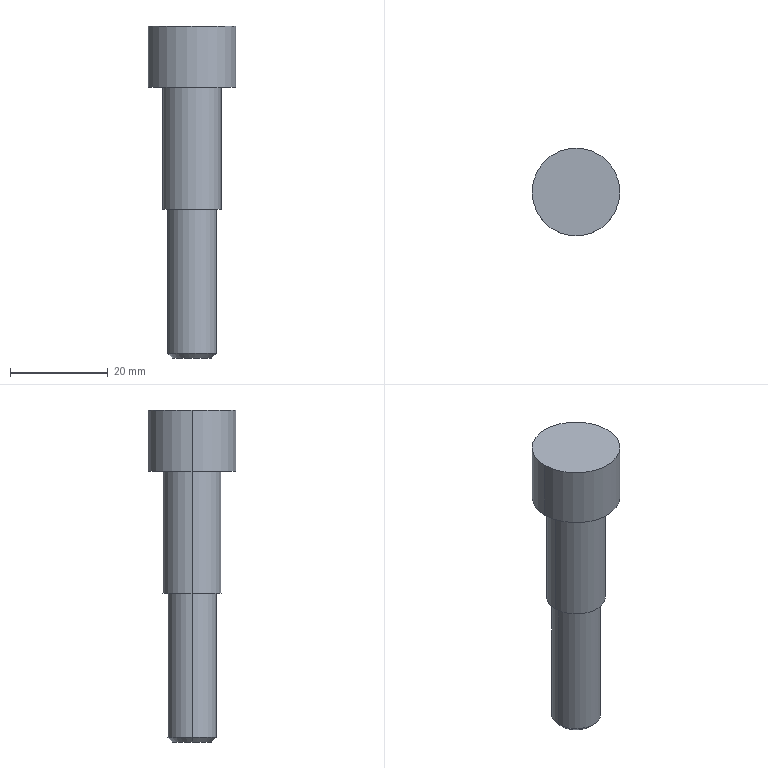Component | SolidWorks | ScrewM10-1 | 1 solid | 12 faces | box 18 x 18 x 68 mm | volume 8389 mm3 | cylinder 6 | plane 4 | cone 2 | commonest cylinder face diameters 10 x2 12 x2 18 x2
build123d program:
from build123d import *

# Parameters (mm, degrees)
CHAMFER1_SIZE = 1


with BuildPart() as part:
    # Sketch1 → Revolve1 (revolve)
    with BuildSketch(Plane.XY, mode=Mode.PRIVATE) as revolve1_sk:
        Polygon((0, 0), (9, 0), (9, 12.5), (6, 12.5), (6, 37.5), (5, 37.5), (5, 68), (0, 68), align=None)
    revolve(revolve1_sk.sketch.rotate(Axis((0, 68, 0), (0, -1, 0)), 180), axis=Axis((0, 68, 0), (0, -1, 0)))

    # Chamfer1
    chamfer1_edges = [part.edges().sort_by_distance(p)[0] for p in [
        (5, 68, 0),
    ]]
    chamfer(chamfer1_edges, length=CHAMFER1_SIZE)


solid = part.part

# Placed as in the assembly
solid = solid.moved(Location((-60.871, 27.262, 12.561), (-90, 0, 0)))
STEP:
#1=CARTESIAN_POINT('',(-2.554,1.073,-2.183));
#2=VERTEX_POINT('',#1);
#3=CARTESIAN_POINT('',(-2.239,1.073,-2.183));
#4=VERTEX_POINT('',#3);
#5=CARTESIAN_POINT('',(-2.396,1.073,-2.183));
#6=DIRECTION('',(0.,-0.,-1.));
#7=DIRECTION('',(1.,0.,0.));
#8=AXIS2_PLACEMENT_3D('',#5,#6,#7);
#9=CIRCLE('',#8,0.1575);
#10=EDGE_CURVE('',#2,#4,#9,.T.);
#11=ORIENTED_EDGE('',*,*,#10,.F.);
#12=CARTESIAN_POINT('',(-2.593,1.073,-2.143));
#13=VERTEX_POINT('',#12);
#14=CARTESIAN_POINT('',(-2.554,1.073,-2.183));
#15=DIRECTION('',(-0.7071,0.,0.7071));
#16=VECTOR('',#15,39.37);
#17=LINE('',#14,#16);
#18=EDGE_CURVE('',#2,#13,#17,.T.);
#19=ORIENTED_EDGE('',*,*,#18,.T.);
#20=CARTESIAN_POINT('',(-2.2,1.073,-2.143));
#21=VERTEX_POINT('',#20);
#22=CARTESIAN_POINT('',(-2.396,1.073,-2.143));
#23=DIRECTION('',(0.,0.,1.));
#24=DIRECTION('',(1.,0.,0.));
#25=AXIS2_PLACEMENT_3D('',#22,#23,#24);
#26=CIRCLE('',#25,0.1969);
#27=EDGE_CURVE('',#21,#13,#26,.T.);
#28=ORIENTED_EDGE('',*,*,#27,.F.);
#29=CARTESIAN_POINT('',(-2.239,1.073,-2.183));
#30=DIRECTION('',(0.7071,0.,0.7071));
#31=VECTOR('',#30,39.37);
#32=LINE('',#29,#31);
#33=EDGE_CURVE('',#4,#21,#32,.T.);
#34=ORIENTED_EDGE('',*,*,#33,.F.);
#35=EDGE_LOOP('',(#11,#19,#28,#34));
#36=FACE_OUTER_BOUND('',#35,.T.);
#37=CARTESIAN_POINT('',(-2.396,1.073,-2.183));
#38=DIRECTION('',(0.,0.,1.));
#39=DIRECTION('',(1.,0.,0.));
#40=AXIS2_PLACEMENT_3D('',#37,#38,#39);
#41=CONICAL_SURFACE('',#40,0.1575,0.7854);
#42=ADVANCED_FACE('',(#36),#41,.T.);
#43=CARTESIAN_POINT('',(-2.593,1.073,-0.9819));
#44=VERTEX_POINT('',#43);
#45=CARTESIAN_POINT('',(-2.2,1.073,-0.9819));
#46=VERTEX_POINT('',#45);
#47=CARTESIAN_POINT('',(-2.396,1.073,-0.9819));
#48=DIRECTION('',(0.,-0.,-1.));
#49=DIRECTION('',(-1.,0.,0.));
#50=AXIS2_PLACEMENT_3D('',#47,#48,#49);
#51=CIRCLE('',#50,0.1969);
#52=EDGE_CURVE('',#44,#46,#51,.T.);
#53=ORIENTED_EDGE('',*,*,#52,.T.);
#54=CARTESIAN_POINT('',(-2.2,1.073,-2.183));
#55=DIRECTION('',(0.,-0.,-1.));
#56=VECTOR('',#55,39.37);
#57=LINE('',#54,#56);
#58=EDGE_CURVE('',#46,#21,#57,.T.);
#59=ORIENTED_EDGE('',*,*,#58,.T.);
#60=ORIENTED_EDGE('',*,*,#27,.T.);
#61=CARTESIAN_POINT('',(-2.593,1.073,-2.183));
#62=DIRECTION('',(0.,-0.,-1.));
#63=VECTOR('',#62,39.37);
#64=LINE('',#61,#63);
#65=EDGE_CURVE('',#44,#13,#64,.T.);
#66=ORIENTED_EDGE('',*,*,#65,.F.);
#67=EDGE_LOOP('',(#53,#59,#60,#66));
#68=FACE_OUTER_BOUND('',#67,.T.);
#69=CARTESIAN_POINT('',(-2.396,1.073,-2.183));
#70=DIRECTION('',(0.,-0.,-1.));
#71=DIRECTION('',(-1.,0.,0.));
#72=AXIS2_PLACEMENT_3D('',#69,#70,#71);
#73=CYLINDRICAL_SURFACE('',#72,0.1969);
#74=ADVANCED_FACE('',(#68),#73,.T.);
#75=CARTESIAN_POINT('',(-2.633,1.073,0.002394));
#76=VERTEX_POINT('',#75);
#77=CARTESIAN_POINT('',(-2.16,1.073,0.002394));
#78=VERTEX_POINT('',#77);
#79=CARTESIAN_POINT('',(-2.396,1.073,0.002394));
#80=DIRECTION('',(0.,-0.,-1.));
#81=DIRECTION('',(-1.,0.,0.));
#82=AXIS2_PLACEMENT_3D('',#79,#80,#81);
#83=CIRCLE('',#82,0.2362);
#84=EDGE_CURVE('',#76,#78,#83,.T.);
#85=ORIENTED_EDGE('',*,*,#84,.T.);
#86=CARTESIAN_POINT('',(-2.16,1.073,-0.9819));
#87=VERTEX_POINT('',#86);
#88=CARTESIAN_POINT('',(-2.16,1.073,-2.183));
#89=DIRECTION('',(0.,-0.,-1.));
#90=VECTOR('',#89,39.37);
#91=LINE('',#88,#90);
#92=EDGE_CURVE('',#78,#87,#91,.T.);
#93=ORIENTED_EDGE('',*,*,#92,.T.);
#94=CARTESIAN_POINT('',(-2.633,1.073,-0.9819));
#95=VERTEX_POINT('',#94);
#96=CARTESIAN_POINT('',(-2.396,1.073,-0.9819));
#97=DIRECTION('',(0.,-0.,-1.));
#98=DIRECTION('',(-1.,0.,0.));
#99=AXIS2_PLACEMENT_3D('',#96,#97,#98);
#100=CIRCLE('',#99,0.2362);
#101=EDGE_CURVE('',#95,#87,#100,.T.);
#102=ORIENTED_EDGE('',*,*,#101,.F.);
#103=CARTESIAN_POINT('',(-2.633,1.073,-2.183));
#104=DIRECTION('',(0.,-0.,-1.));
#105=VECTOR('',#104,39.37);
#106=LINE('',#103,#105);
#107=EDGE_CURVE('',#76,#95,#106,.T.);
#108=ORIENTED_EDGE('',*,*,#107,.F.);
#109=EDGE_LOOP('',(#85,#93,#102,#108));
#110=FACE_OUTER_BOUND('',#109,.T.);
#111=CARTESIAN_POINT('',(-2.396,1.073,-2.183));
#112=DIRECTION('',(0.,-0.,-1.));
#113=DIRECTION('',(-1.,0.,0.));
#114=AXIS2_PLACEMENT_3D('',#111,#112,#113);
#115=CYLINDRICAL_SURFACE('',#114,0.2362);
#116=ADVANCED_FACE('',(#110),#115,.T.);
#117=CARTESIAN_POINT('',(-2.751,1.073,0.4945));
#118=VERTEX_POINT('',#117);
#119=CARTESIAN_POINT('',(-2.042,1.073,0.4945));
#120=VERTEX_POINT('',#119);
#121=CARTESIAN_POINT('',(-2.396,1.073,0.4945));
#122=DIRECTION('',(0.,-0.,-1.));
#123=DIRECTION('',(-1.,0.,0.));
#124=AXIS2_PLACEMENT_3D('',#121,#122,#123);
#125=CIRCLE('',#124,0.3543);
#126=EDGE_CURVE('',#118,#120,#125,.T.);
#127=ORIENTED_EDGE('',*,*,#126,.T.);
#128=CARTESIAN_POINT('',(-2.042,1.073,0.002394));
#129=VERTEX_POINT('',#128);
#130=CARTESIAN_POINT('',(-2.042,1.073,-2.183));
#131=DIRECTION('',(0.,-0.,-1.));
#132=VECTOR('',#131,39.37);
#133=LINE('',#130,#132);
#134=EDGE_CURVE('',#120,#129,#133,.T.);
#135=ORIENTED_EDGE('',*,*,#134,.T.);
#136=CARTESIAN_POINT('',(-2.751,1.073,0.002394));
#137=VERTEX_POINT('',#136);
#138=CARTESIAN_POINT('',(-2.396,1.073,0.002394));
#139=DIRECTION('',(0.,-0.,-1.));
#140=DIRECTION('',(-1.,0.,0.));
#141=AXIS2_PLACEMENT_3D('',#138,#139,#140);
#142=CIRCLE('',#141,0.3543);
#143=EDGE_CURVE('',#137,#129,#142,.T.);
#144=ORIENTED_EDGE('',*,*,#143,.F.);
#145=CARTESIAN_POINT('',(-2.751,1.073,-2.183));
#146=DIRECTION('',(0.,-0.,-1.));
#147=VECTOR('',#146,39.37);
#148=LINE('',#145,#147);
#149=EDGE_CURVE('',#118,#137,#148,.T.);
#150=ORIENTED_EDGE('',*,*,#149,.F.);
#151=EDGE_LOOP('',(#127,#135,#144,#150));
#152=FACE_OUTER_BOUND('',#151,.T.);
#153=CARTESIAN_POINT('',(-2.396,1.073,-2.183));
#154=DIRECTION('',(0.,-0.,-1.));
#155=DIRECTION('',(-1.,0.,0.));
#156=AXIS2_PLACEMENT_3D('',#153,#154,#155);
#157=CYLINDRICAL_SURFACE('',#156,0.3543);
#158=ADVANCED_FACE('',(#152),#157,.T.);
#159=ORIENTED_EDGE('',*,*,#126,.F.);
#160=CARTESIAN_POINT('',(-2.396,1.073,0.4945));
#161=DIRECTION('',(0.,-0.,-1.));
#162=DIRECTION('',(-1.,0.,0.));
#163=AXIS2_PLACEMENT_3D('',#160,#161,#162);
#164=CIRCLE('',#163,0.3543);
#165=EDGE_CURVE('',#120,#118,#164,.T.);
#166=ORIENTED_EDGE('',*,*,#165,.F.);
#167=EDGE_LOOP('',(#159,#166));
#168=FACE_OUTER_BOUND('',#167,.T.);
#169=CARTESIAN_POINT('',(-2.396,1.073,0.4945));
#170=DIRECTION('',(0.,-0.,-1.));
#171=DIRECTION('',(-1.,-0.,0.));
#172=AXIS2_PLACEMENT_3D('',#169,#170,#171);
#173=PLANE('',#172);
#174=ADVANCED_FACE('',(#168),#173,.F.);
#175=ORIENTED_EDGE('',*,*,#134,.F.);
#176=ORIENTED_EDGE('',*,*,#165,.T.);
#177=ORIENTED_EDGE('',*,*,#149,.T.);
#178=CARTESIAN_POINT('',(-2.396,1.073,0.002394));
#179=DIRECTION('',(0.,-0.,-1.));
#180=DIRECTION('',(-1.,0.,0.));
#181=AXIS2_PLACEMENT_3D('',#178,#179,#180);
#182=CIRCLE('',#181,0.3543);
#183=EDGE_CURVE('',#129,#137,#182,.T.);
#184=ORIENTED_EDGE('',*,*,#183,.F.);
#185=EDGE_LOOP('',(#175,#176,#177,#184));
#186=FACE_OUTER_BOUND('',#185,.T.);
#187=CARTESIAN_POINT('',(-2.396,1.073,-2.183));
#188=DIRECTION('',(0.,-0.,-1.));
#189=DIRECTION('',(-1.,0.,0.));
#190=AXIS2_PLACEMENT_3D('',#187,#188,#189);
#191=CYLINDRICAL_SURFACE('',#190,0.3543);
#192=ADVANCED_FACE('',(#186),#191,.T.);
#193=ORIENTED_EDGE('',*,*,#84,.F.);
#194=CARTESIAN_POINT('',(-2.396,1.073,0.002394));
#195=DIRECTION('',(0.,-0.,-1.));
#196=DIRECTION('',(-1.,0.,0.));
#197=AXIS2_PLACEMENT_3D('',#194,#195,#196);
#198=CIRCLE('',#197,0.2362);
#199=EDGE_CURVE('',#78,#76,#198,.T.);
#200=ORIENTED_EDGE('',*,*,#199,.F.);
#201=EDGE_LOOP('',(#193,#200));
#202=FACE_BOUND('',#201,.T.);
#203=ORIENTED_EDGE('',*,*,#143,.T.);
#204=ORIENTED_EDGE('',*,*,#183,.T.);
#205=EDGE_LOOP('',(#203,#204));
#206=FACE_OUTER_BOUND('',#205,.T.);
#207=CARTESIAN_POINT('',(-2.042,1.073,0.002394));
#208=DIRECTION('',(-0.,0.,1.));
#209=DIRECTION('',(1.,0.,0.));
#210=AXIS2_PLACEMENT_3D('',#207,#208,#209);
#211=PLANE('',#210);
#212=ADVANCED_FACE('',(#202,#206),#211,.F.);
#213=ORIENTED_EDGE('',*,*,#92,.F.);
#214=ORIENTED_EDGE('',*,*,#199,.T.);
#215=ORIENTED_EDGE('',*,*,#107,.T.);
#216=CARTESIAN_POINT('',(-2.396,1.073,-0.9819));
#217=DIRECTION('',(0.,-0.,-1.));
#218=DIRECTION('',(-1.,0.,0.));
#219=AXIS2_PLACEMENT_3D('',#216,#217,#218);
#220=CIRCLE('',#219,0.2362);
#221=EDGE_CURVE('',#87,#95,#220,.T.);
#222=ORIENTED_EDGE('',*,*,#221,.F.);
#223=EDGE_LOOP('',(#213,#214,#215,#222));
#224=FACE_OUTER_BOUND('',#223,.T.);
#225=CARTESIAN_POINT('',(-2.396,1.073,-2.183));
#226=DIRECTION('',(0.,-0.,-1.));
#227=DIRECTION('',(-1.,0.,0.));
#228=AXIS2_PLACEMENT_3D('',#225,#226,#227);
#229=CYLINDRICAL_SURFACE('',#228,0.2362);
#230=ADVANCED_FACE('',(#224),#229,.T.);
#231=ORIENTED_EDGE('',*,*,#52,.F.);
#232=CARTESIAN_POINT('',(-2.396,1.073,-0.9819));
#233=DIRECTION('',(0.,-0.,-1.));
#234=DIRECTION('',(-1.,0.,0.));
#235=AXIS2_PLACEMENT_3D('',#232,#233,#234);
#236=CIRCLE('',#235,0.1969);
#237=EDGE_CURVE('',#46,#44,#236,.T.);
#238=ORIENTED_EDGE('',*,*,#237,.F.);
#239=EDGE_LOOP('',(#231,#238));
#240=FACE_BOUND('',#239,.T.);
#241=ORIENTED_EDGE('',*,*,#101,.T.);
#242=ORIENTED_EDGE('',*,*,#221,.T.);
#243=EDGE_LOOP('',(#241,#242));
#244=FACE_OUTER_BOUND('',#243,.T.);
#245=CARTESIAN_POINT('',(-2.16,1.073,-0.9819));
#246=DIRECTION('',(-0.,0.,1.));
#247=DIRECTION('',(1.,0.,0.));
#248=AXIS2_PLACEMENT_3D('',#245,#246,#247);
#249=PLANE('',#248);
#250=ADVANCED_FACE('',(#240,#244),#249,.F.);
#251=ORIENTED_EDGE('',*,*,#58,.F.);
#252=ORIENTED_EDGE('',*,*,#237,.T.);
#253=ORIENTED_EDGE('',*,*,#65,.T.);
#254=CARTESIAN_POINT('',(-2.396,1.073,-2.143));
#255=DIRECTION('',(0.,0.,1.));
#256=DIRECTION('',(1.,0.,0.));
#257=AXIS2_PLACEMENT_3D('',#254,#255,#256);
#258=CIRCLE('',#257,0.1969);
#259=EDGE_CURVE('',#13,#21,#258,.T.);
#260=ORIENTED_EDGE('',*,*,#259,.T.);
#261=EDGE_LOOP('',(#251,#252,#253,#260));
#262=FACE_OUTER_BOUND('',#261,.T.);
#263=CARTESIAN_POINT('',(-2.396,1.073,-2.183));
#264=DIRECTION('',(0.,-0.,-1.));
#265=DIRECTION('',(-1.,0.,0.));
#266=AXIS2_PLACEMENT_3D('',#263,#264,#265);
#267=CYLINDRICAL_SURFACE('',#266,0.1969);
#268=ADVANCED_FACE('',(#262),#267,.T.);
#269=CARTESIAN_POINT('',(-2.396,1.073,-2.183));
#270=DIRECTION('',(0.,-0.,-1.));
#271=DIRECTION('',(1.,0.,0.));
#272=AXIS2_PLACEMENT_3D('',#269,#270,#271);
#273=CIRCLE('',#272,0.1575);
#274=EDGE_CURVE('',#4,#2,#273,.T.);
#275=ORIENTED_EDGE('',*,*,#274,.T.);
#276=ORIENTED_EDGE('',*,*,#10,.T.);
#277=EDGE_LOOP('',(#275,#276));
#278=FACE_OUTER_BOUND('',#277,.T.);
#279=CARTESIAN_POINT('',(-2.2,1.073,-2.183));
#280=DIRECTION('',(-0.,0.,1.));
#281=DIRECTION('',(1.,0.,0.));
#282=AXIS2_PLACEMENT_3D('',#279,#280,#281);
#283=PLANE('',#282);
#284=ADVANCED_FACE('',(#278),#283,.F.);
#285=ORIENTED_EDGE('',*,*,#18,.F.);
#286=ORIENTED_EDGE('',*,*,#274,.F.);
#287=ORIENTED_EDGE('',*,*,#33,.T.);
#288=ORIENTED_EDGE('',*,*,#259,.F.);
#289=EDGE_LOOP('',(#285,#286,#287,#288));
#290=FACE_OUTER_BOUND('',#289,.T.);
#291=CARTESIAN_POINT('',(-2.396,1.073,-2.183));
#292=DIRECTION('',(0.,0.,1.));
#293=DIRECTION('',(1.,0.,0.));
#294=AXIS2_PLACEMENT_3D('',#291,#292,#293);
#295=CONICAL_SURFACE('',#294,0.1575,0.7854);
#296=ADVANCED_FACE('',(#290),#295,.T.);
#297=CLOSED_SHELL('',(#42,#74,#116,#158,#174,#192,#212,#230,#250,#268,#284,#296));
#298=MANIFOLD_SOLID_BREP('',#297);
#299=CARTESIAN_POINT('',(0.,0.,0.));
#300=DIRECTION('',(0.,0.,1.));
#301=DIRECTION('',(1.,0.,0.));
#302=AXIS2_PLACEMENT_3D('',#299,#300,#301);
#303=(LENGTH_UNIT()NAMED_UNIT(*)SI_UNIT($,.METRE.));
#304=LENGTH_MEASURE_WITH_UNIT(LENGTH_MEASURE(0.0254),#303);
#305=DIMENSIONAL_EXPONENTS(1.,0.,0.,0.,0.,0.,0.);
#306=(CONVERSION_BASED_UNIT('',#304)LENGTH_UNIT()NAMED_UNIT(#305));
#307=UNCERTAINTY_MEASURE_WITH_UNIT(LENGTH_MEASURE(0.00001),#306,'','');
#308=(NAMED_UNIT(*)PLANE_ANGLE_UNIT()SI_UNIT($,.RADIAN.));
#309=(NAMED_UNIT(*)SI_UNIT($,.STERADIAN.)SOLID_ANGLE_UNIT());
#310=(GEOMETRIC_REPRESENTATION_CONTEXT(3)GLOBAL_UNCERTAINTY_ASSIGNED_CONTEXT((#307))GLOBAL_UNIT_ASSIGNED_CONTEXT((#306,#308,#309))REPRESENTATION_CONTEXT('',''));
#311=ADVANCED_BREP_SHAPE_REPRESENTATION('',(#298,#302),#310);
#312=COLOUR_RGB('',0.7922,0.8196,0.9333);
#313=FILL_AREA_STYLE_COLOUR('',#312);
#314=FILL_AREA_STYLE('',(#313));
#315=SURFACE_STYLE_FILL_AREA(#314);
#316=SURFACE_SIDE_STYLE('',(#315));
#317=SURFACE_STYLE_USAGE(.BOTH.,#316);
#318=PRESENTATION_STYLE_ASSIGNMENT((#317));
#319=STYLED_ITEM('',(#318),#298);
#320=(LENGTH_UNIT()NAMED_UNIT(*)SI_UNIT($,.METRE.));
#321=LENGTH_MEASURE_WITH_UNIT(LENGTH_MEASURE(0.0254),#320);
#322=DIMENSIONAL_EXPONENTS(1.,0.,0.,0.,0.,0.,0.);
#323=(CONVERSION_BASED_UNIT('',#321)LENGTH_UNIT()NAMED_UNIT(#322));
#324=UNCERTAINTY_MEASURE_WITH_UNIT(LENGTH_MEASURE(0.00001),#323,'','');
#325=(NAMED_UNIT(*)PLANE_ANGLE_UNIT()SI_UNIT($,.RADIAN.));
#326=(NAMED_UNIT(*)SI_UNIT($,.STERADIAN.)SOLID_ANGLE_UNIT());
#327=(GEOMETRIC_REPRESENTATION_CONTEXT(3)GLOBAL_UNCERTAINTY_ASSIGNED_CONTEXT((#324))GLOBAL_UNIT_ASSIGNED_CONTEXT((#323,#325,#326))REPRESENTATION_CONTEXT('',''));
#328=MECHANICAL_DESIGN_GEOMETRIC_PRESENTATION_REPRESENTATION('',(#319),#327);
#329=PRESENTATION_LAYER_ASSIGNMENT('','',(#319));